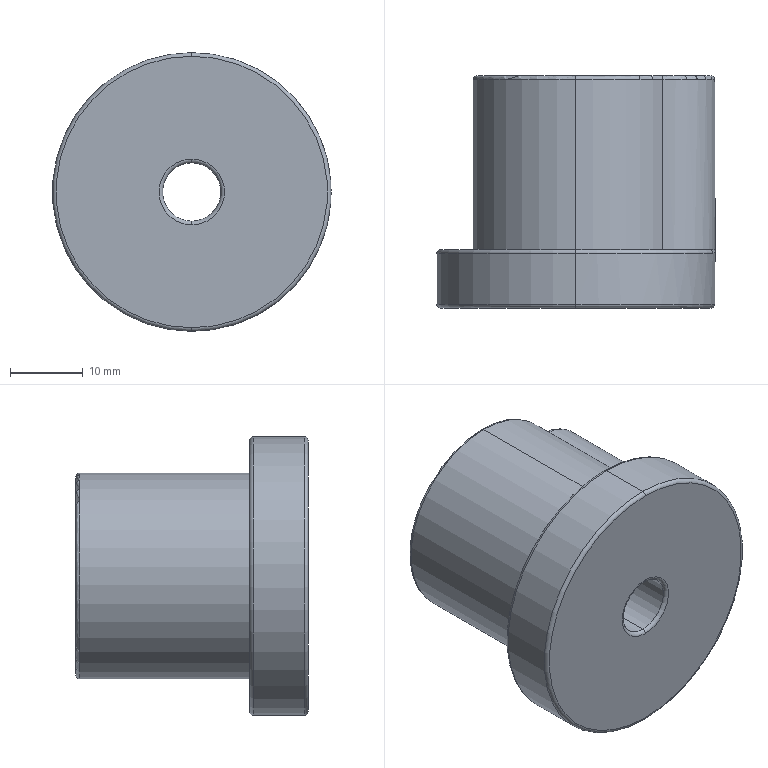Component | SolidWorks | Workpiece-1 | 1 solid | 26 faces | box 38.21 x 31.82 x 38.21 mm | volume 23902 mm3 | torus 13 | cylinder 8 | plane 3 | spline 2 | commonest cylinder face diameters 28.21 x3 38.21 x2 8 x2 15 x1 | material 45
STEP:
#1=COLOUR_RGB('',0.7922,0.8196,0.9333);
#2=FILL_AREA_STYLE_COLOUR('',#1);
#3=FILL_AREA_STYLE('',(#2));
#4=SURFACE_STYLE_FILL_AREA(#3);
#5=SURFACE_SIDE_STYLE('',(#4));
#6=SURFACE_STYLE_USAGE(.BOTH.,#5);
#7=PRESENTATION_STYLE_ASSIGNMENT((#6));
#8=CARTESIAN_POINT('',(-14.62,-0.1144,42.544));
#9=VERTEX_POINT('',#8);
#10=CARTESIAN_POINT('',(-13.9,-0.1144,41.945));
#11=VERTEX_POINT('',#10);
#12=CARTESIAN_POINT('',(-14.62,-0.1144,41.811));
#13=DIRECTION('',(0.,1.,0.));
#14=DIRECTION('',(-0.,0.,-1.));
#15=AXIS2_PLACEMENT_3D('',#12,#13,#14);
#16=CIRCLE('',#15,0.7325);
#17=EDGE_CURVE('',#9,#11,#16,.T.);
#18=ORIENTED_EDGE('',*,*,#17,.F.);
#19=CARTESIAN_POINT('',(-14.62,-0.1341,42.563));
#20=VERTEX_POINT('',#19);
#21=CARTESIAN_POINT('',(-14.62,-0.1341,42.544));
#22=DIRECTION('',(1.,0.,-0.));
#23=DIRECTION('',(0.,0.,-1.));
#24=AXIS2_PLACEMENT_3D('',#21,#22,#23);
#25=CIRCLE('',#24,0.01969);
#26=EDGE_CURVE('',#9,#20,#25,.T.);
#27=ORIENTED_EDGE('',*,*,#26,.T.);
#28=CARTESIAN_POINT('',(-13.881,-0.1341,41.948));
#29=VERTEX_POINT('',#28);
#30=CARTESIAN_POINT('',(-14.62,-0.1341,41.811));
#31=DIRECTION('',(0.,-1.,0.));
#32=DIRECTION('',(0.,0.,-1.));
#33=AXIS2_PLACEMENT_3D('',#30,#31,#32);
#34=CIRCLE('',#33,0.7522);
#35=EDGE_CURVE('',#29,#20,#34,.T.);
#36=ORIENTED_EDGE('',*,*,#35,.F.);
#37=CARTESIAN_POINT('',(-13.9,-0.1341,41.945));
#38=DIRECTION('',(0.1825,0.,-0.9832));
#39=DIRECTION('',(-0.9832,0.,-0.1825));
#40=AXIS2_PLACEMENT_3D('',#37,#38,#39);
#41=CIRCLE('',#40,0.01969);
#42=EDGE_CURVE('',#11,#29,#41,.T.);
#43=ORIENTED_EDGE('',*,*,#42,.F.);
#44=EDGE_LOOP('',(#18,#27,#36,#43));
#45=FACE_OUTER_BOUND('',#44,.T.);
#46=CARTESIAN_POINT('',(-14.62,-0.1341,41.811));
#47=DIRECTION('',(0.,-1.,0.));
#48=DIRECTION('',(0.,0.,-1.));
#49=AXIS2_PLACEMENT_3D('',#46,#47,#48);
#50=TOROIDAL_SURFACE('',#49,0.7325,0.01969);
#51=ADVANCED_FACE('',(#45),#50,.T.);
#52=ORIENTED_EDGE('',*,*,#26,.F.);
#53=CARTESIAN_POINT('',(-14.62,-0.1144,41.079));
#54=VERTEX_POINT('',#53);
#55=CARTESIAN_POINT('',(-14.62,-0.1144,41.811));
#56=DIRECTION('',(0.,1.,0.));
#57=DIRECTION('',(0.,0.,-1.));
#58=AXIS2_PLACEMENT_3D('',#55,#56,#57);
#59=CIRCLE('',#58,0.7325);
#60=EDGE_CURVE('',#54,#9,#59,.T.);
#61=ORIENTED_EDGE('',*,*,#60,.F.);
#62=CARTESIAN_POINT('',(-14.62,-0.1341,41.059));
#63=VERTEX_POINT('',#62);
#64=CARTESIAN_POINT('',(-14.62,-0.1341,41.079));
#65=DIRECTION('',(-1.,0.,0.));
#66=DIRECTION('',(0.,0.,1.));
#67=AXIS2_PLACEMENT_3D('',#64,#65,#66);
#68=CIRCLE('',#67,0.01969);
#69=EDGE_CURVE('',#54,#63,#68,.T.);
#70=ORIENTED_EDGE('',*,*,#69,.T.);
#71=CARTESIAN_POINT('',(-14.62,-0.1341,41.811));
#72=DIRECTION('',(0.,-1.,0.));
#73=DIRECTION('',(0.,0.,-1.));
#74=AXIS2_PLACEMENT_3D('',#71,#72,#73);
#75=CIRCLE('',#74,0.7522);
#76=EDGE_CURVE('',#20,#63,#75,.T.);
#77=ORIENTED_EDGE('',*,*,#76,.F.);
#78=EDGE_LOOP('',(#52,#61,#70,#77));
#79=FACE_OUTER_BOUND('',#78,.T.);
#80=CARTESIAN_POINT('',(-14.62,-0.1341,41.811));
#81=DIRECTION('',(0.,-1.,0.));
#82=DIRECTION('',(0.,0.,-1.));
#83=AXIS2_PLACEMENT_3D('',#80,#81,#82);
#84=TOROIDAL_SURFACE('',#83,0.7325,0.01969);
#85=ADVANCED_FACE('',(#79),#84,.T.);
#86=CARTESIAN_POINT('',(-14.62,0.8037,41.256));
#87=VERTEX_POINT('',#86);
#88=CARTESIAN_POINT('',(-14.15,0.8037,41.516));
#89=VERTEX_POINT('',#88);
#90=CARTESIAN_POINT('',(-14.62,0.8037,41.811));
#91=DIRECTION('',(0.,-1.,0.));
#92=DIRECTION('',(-0.,0.,1.));
#93=AXIS2_PLACEMENT_3D('',#90,#91,#92);
#94=CIRCLE('',#93,0.5553);
#95=EDGE_CURVE('',#87,#89,#94,.T.);
#96=ORIENTED_EDGE('',*,*,#95,.F.);
#97=CARTESIAN_POINT('',(-14.62,0.8234,41.275));
#98=VERTEX_POINT('',#97);
#99=CARTESIAN_POINT('',(-14.62,0.8037,41.275));
#100=DIRECTION('',(1.,0.,0.));
#101=DIRECTION('',(0.,0.,-1.));
#102=AXIS2_PLACEMENT_3D('',#99,#100,#101);
#103=CIRCLE('',#102,0.01969);
#104=EDGE_CURVE('',#87,#98,#103,.T.);
#105=ORIENTED_EDGE('',*,*,#104,.T.);
#106=CARTESIAN_POINT('',(-14.161,0.8234,41.535));
#107=VERTEX_POINT('',#106);
#108=CARTESIAN_POINT('',(-14.62,0.8234,41.811));
#109=DIRECTION('',(0.,1.,0.));
#110=DIRECTION('',(0.,0.,1.));
#111=AXIS2_PLACEMENT_3D('',#108,#109,#110);
#112=CIRCLE('',#111,0.5356);
#113=EDGE_CURVE('',#107,#98,#112,.T.);
#114=ORIENTED_EDGE('',*,*,#113,.F.);
#115=CARTESIAN_POINT('',(-14.15,0.8037,41.516));
#116=CARTESIAN_POINT('',(-14.15,0.8093,41.516));
#117=CARTESIAN_POINT('',(-14.151,0.8146,41.518));
#118=CARTESIAN_POINT('',(-14.156,0.8216,41.526));
#119=CARTESIAN_POINT('',(-14.158,0.8234,41.531));
#120=CARTESIAN_POINT('',(-14.161,0.8234,41.535));
#121=B_SPLINE_CURVE_WITH_KNOTS('',3,(#115,#116,#117,#118,#119,#120),.UNSPECIFIED.,.F.,.F.,(4,2,4),(0.,0.0004181,0.0008363),.UNSPECIFIED.);
#122=EDGE_CURVE('',#89,#107,#121,.T.);
#123=ORIENTED_EDGE('',*,*,#122,.F.);
#124=EDGE_LOOP('',(#96,#105,#114,#123));
#125=FACE_OUTER_BOUND('',#124,.T.);
#126=CARTESIAN_POINT('',(-14.62,0.8037,41.811));
#127=DIRECTION('',(0.,1.,0.));
#128=DIRECTION('',(0.,0.,1.));
#129=AXIS2_PLACEMENT_3D('',#126,#127,#128);
#130=TOROIDAL_SURFACE('',#129,0.5356,0.01969);
#131=ADVANCED_FACE('',(#125),#130,.T.);
#132=ORIENTED_EDGE('',*,*,#104,.F.);
#133=CARTESIAN_POINT('',(-14.62,0.8037,42.366));
#134=VERTEX_POINT('',#133);
#135=CARTESIAN_POINT('',(-14.62,0.8037,41.811));
#136=DIRECTION('',(0.,-1.,0.));
#137=DIRECTION('',(0.,0.,1.));
#138=AXIS2_PLACEMENT_3D('',#135,#136,#137);
#139=CIRCLE('',#138,0.5553);
#140=EDGE_CURVE('',#134,#87,#139,.T.);
#141=ORIENTED_EDGE('',*,*,#140,.F.);
#142=CARTESIAN_POINT('',(-14.62,0.8234,42.347));
#143=VERTEX_POINT('',#142);
#144=CARTESIAN_POINT('',(-14.62,0.8037,42.347));
#145=DIRECTION('',(-1.,0.,0.));
#146=DIRECTION('',(0.,0.,1.));
#147=AXIS2_PLACEMENT_3D('',#144,#145,#146);
#148=CIRCLE('',#147,0.01969);
#149=EDGE_CURVE('',#134,#143,#148,.T.);
#150=ORIENTED_EDGE('',*,*,#149,.T.);
#151=CARTESIAN_POINT('',(-14.62,0.8234,41.811));
#152=DIRECTION('',(0.,1.,0.));
#153=DIRECTION('',(0.,0.,1.));
#154=AXIS2_PLACEMENT_3D('',#151,#152,#153);
#155=CIRCLE('',#154,0.5356);
#156=EDGE_CURVE('',#98,#143,#155,.T.);
#157=ORIENTED_EDGE('',*,*,#156,.F.);
#158=EDGE_LOOP('',(#132,#141,#150,#157));
#159=FACE_OUTER_BOUND('',#158,.T.);
#160=CARTESIAN_POINT('',(-14.62,0.8037,41.811));
#161=DIRECTION('',(0.,1.,0.));
#162=DIRECTION('',(0.,0.,1.));
#163=AXIS2_PLACEMENT_3D('',#160,#161,#162);
#164=TOROIDAL_SURFACE('',#163,0.5356,0.01969);
#165=ADVANCED_FACE('',(#159),#164,.T.);
#166=CARTESIAN_POINT('',(-14.62,0.8234,41.634));
#167=VERTEX_POINT('',#166);
#168=CARTESIAN_POINT('',(-14.62,0.8234,41.988));
#169=VERTEX_POINT('',#168);
#170=CARTESIAN_POINT('',(-14.62,0.8234,41.811));
#171=DIRECTION('',(0.,-1.,0.));
#172=DIRECTION('',(0.,0.,1.));
#173=AXIS2_PLACEMENT_3D('',#170,#171,#172);
#174=CIRCLE('',#173,0.1772);
#175=EDGE_CURVE('',#167,#169,#174,.T.);
#176=ORIENTED_EDGE('',*,*,#175,.F.);
#177=CARTESIAN_POINT('',(-14.62,0.8037,41.654));
#178=VERTEX_POINT('',#177);
#179=CARTESIAN_POINT('',(-14.62,0.8037,41.634));
#180=DIRECTION('',(1.,0.,0.));
#181=DIRECTION('',(0.,0.,-1.));
#182=AXIS2_PLACEMENT_3D('',#179,#180,#181);
#183=CIRCLE('',#182,0.01969);
#184=EDGE_CURVE('',#167,#178,#183,.T.);
#185=ORIENTED_EDGE('',*,*,#184,.T.);
#186=CARTESIAN_POINT('',(-14.62,0.8037,41.969));
#187=VERTEX_POINT('',#186);
#188=CARTESIAN_POINT('',(-14.62,0.8037,41.811));
#189=DIRECTION('',(0.,1.,0.));
#190=DIRECTION('',(0.,0.,1.));
#191=AXIS2_PLACEMENT_3D('',#188,#189,#190);
#192=CIRCLE('',#191,0.1575);
#193=EDGE_CURVE('',#187,#178,#192,.T.);
#194=ORIENTED_EDGE('',*,*,#193,.F.);
#195=CARTESIAN_POINT('',(-14.62,0.8037,41.988));
#196=DIRECTION('',(-1.,0.,0.));
#197=DIRECTION('',(0.,0.,1.));
#198=AXIS2_PLACEMENT_3D('',#195,#196,#197);
#199=CIRCLE('',#198,0.01969);
#200=EDGE_CURVE('',#169,#187,#199,.T.);
#201=ORIENTED_EDGE('',*,*,#200,.F.);
#202=EDGE_LOOP('',(#176,#185,#194,#201));
#203=FACE_OUTER_BOUND('',#202,.T.);
#204=CARTESIAN_POINT('',(-14.62,0.8037,41.811));
#205=DIRECTION('',(0.,1.,0.));
#206=DIRECTION('',(0.,0.,1.));
#207=AXIS2_PLACEMENT_3D('',#204,#205,#206);
#208=TOROIDAL_SURFACE('',#207,0.1772,0.01969);
#209=ADVANCED_FACE('',(#203),#208,.T.);
#210=CARTESIAN_POINT('',(-14.62,-0.4097,42.563));
#211=VERTEX_POINT('',#210);
#212=CARTESIAN_POINT('',(-14.62,-0.4097,41.059));
#213=VERTEX_POINT('',#212);
#214=CARTESIAN_POINT('',(-14.62,-0.4097,41.811));
#215=DIRECTION('',(0.,1.,0.));
#216=DIRECTION('',(0.,0.,-1.));
#217=AXIS2_PLACEMENT_3D('',#214,#215,#216);
#218=CIRCLE('',#217,0.7522);
#219=EDGE_CURVE('',#211,#213,#218,.T.);
#220=ORIENTED_EDGE('',*,*,#219,.F.);
#221=CARTESIAN_POINT('',(-14.62,-0.4293,42.544));
#222=VERTEX_POINT('',#221);
#223=CARTESIAN_POINT('',(-14.62,-0.4097,42.544));
#224=DIRECTION('',(1.,0.,-0.));
#225=DIRECTION('',(0.,0.,-1.));
#226=AXIS2_PLACEMENT_3D('',#223,#224,#225);
#227=CIRCLE('',#226,0.01969);
#228=EDGE_CURVE('',#211,#222,#227,.T.);
#229=ORIENTED_EDGE('',*,*,#228,.T.);
#230=CARTESIAN_POINT('',(-14.62,-0.4293,41.079));
#231=VERTEX_POINT('',#230);
#232=CARTESIAN_POINT('',(-14.62,-0.4293,41.811));
#233=DIRECTION('',(0.,-1.,0.));
#234=DIRECTION('',(0.,0.,-1.));
#235=AXIS2_PLACEMENT_3D('',#232,#233,#234);
#236=CIRCLE('',#235,0.7325);
#237=EDGE_CURVE('',#231,#222,#236,.T.);
#238=ORIENTED_EDGE('',*,*,#237,.F.);
#239=CARTESIAN_POINT('',(-14.62,-0.4097,41.079));
#240=DIRECTION('',(-1.,0.,0.));
#241=DIRECTION('',(0.,0.,1.));
#242=AXIS2_PLACEMENT_3D('',#239,#240,#241);
#243=CIRCLE('',#242,0.01969);
#244=EDGE_CURVE('',#213,#231,#243,.T.);
#245=ORIENTED_EDGE('',*,*,#244,.F.);
#246=EDGE_LOOP('',(#220,#229,#238,#245));
#247=FACE_OUTER_BOUND('',#246,.T.);
#248=CARTESIAN_POINT('',(-14.62,-0.4097,41.811));
#249=DIRECTION('',(0.,-1.,0.));
#250=DIRECTION('',(0.,0.,-1.));
#251=AXIS2_PLACEMENT_3D('',#248,#249,#250);
#252=TOROIDAL_SURFACE('',#251,0.7325,0.01969);
#253=ADVANCED_FACE('',(#247),#252,.T.);
#254=CARTESIAN_POINT('',(-14.62,-0.4293,41.988));
#255=VERTEX_POINT('',#254);
#256=CARTESIAN_POINT('',(-14.62,-0.4293,41.634));
#257=VERTEX_POINT('',#256);
#258=CARTESIAN_POINT('',(-14.62,-0.4293,41.811));
#259=DIRECTION('',(0.,1.,0.));
#260=DIRECTION('',(0.,0.,-1.));
#261=AXIS2_PLACEMENT_3D('',#258,#259,#260);
#262=CIRCLE('',#261,0.1772);
#263=EDGE_CURVE('',#255,#257,#262,.T.);
#264=ORIENTED_EDGE('',*,*,#263,.F.);
#265=CARTESIAN_POINT('',(-14.62,-0.4097,41.969));
#266=VERTEX_POINT('',#265);
#267=CARTESIAN_POINT('',(-14.62,-0.4097,41.988));
#268=DIRECTION('',(1.,0.,-0.));
#269=DIRECTION('',(0.,0.,-1.));
#270=AXIS2_PLACEMENT_3D('',#267,#268,#269);
#271=CIRCLE('',#270,0.01969);
#272=EDGE_CURVE('',#255,#266,#271,.T.);
#273=ORIENTED_EDGE('',*,*,#272,.T.);
#274=CARTESIAN_POINT('',(-14.62,-0.4097,41.654));
#275=VERTEX_POINT('',#274);
#276=CARTESIAN_POINT('',(-14.62,-0.4097,41.811));
#277=DIRECTION('',(0.,-1.,0.));
#278=DIRECTION('',(0.,0.,-1.));
#279=AXIS2_PLACEMENT_3D('',#276,#277,#278);
#280=CIRCLE('',#279,0.1575);
#281=EDGE_CURVE('',#275,#266,#280,.T.);
#282=ORIENTED_EDGE('',*,*,#281,.F.);
#283=CARTESIAN_POINT('',(-14.62,-0.4097,41.634));
#284=DIRECTION('',(-1.,0.,0.));
#285=DIRECTION('',(0.,0.,1.));
#286=AXIS2_PLACEMENT_3D('',#283,#284,#285);
#287=CIRCLE('',#286,0.01969);
#288=EDGE_CURVE('',#257,#275,#287,.T.);
#289=ORIENTED_EDGE('',*,*,#288,.F.);
#290=EDGE_LOOP('',(#264,#273,#282,#289));
#291=FACE_OUTER_BOUND('',#290,.T.);
#292=CARTESIAN_POINT('',(-14.62,-0.4097,41.811));
#293=DIRECTION('',(0.,-1.,0.));
#294=DIRECTION('',(0.,0.,-1.));
#295=AXIS2_PLACEMENT_3D('',#292,#293,#294);
#296=TOROIDAL_SURFACE('',#295,0.1772,0.01969);
#297=ADVANCED_FACE('',(#291),#296,.T.);
#298=ORIENTED_EDGE('',*,*,#219,.T.);
#299=CARTESIAN_POINT('',(-14.62,-0.4293,41.059));
#300=DIRECTION('',(0.,1.,0.));
#301=VECTOR('',#300,39.37);
#302=LINE('',#299,#301);
#303=EDGE_CURVE('',#213,#63,#302,.T.);
#304=ORIENTED_EDGE('',*,*,#303,.T.);
#305=CARTESIAN_POINT('',(-13.881,-0.1341,41.674));
#306=VERTEX_POINT('',#305);
#307=CARTESIAN_POINT('',(-14.62,-0.1341,41.811));
#308=DIRECTION('',(0.,-1.,0.));
#309=DIRECTION('',(0.,0.,-1.));
#310=AXIS2_PLACEMENT_3D('',#307,#308,#309);
#311=CIRCLE('',#310,0.7522);
#312=EDGE_CURVE('',#63,#306,#311,.T.);
#313=ORIENTED_EDGE('',*,*,#312,.T.);
#314=CARTESIAN_POINT('',(-13.868,-0.1144,41.811));
#315=VERTEX_POINT('',#314);
#316=CARTESIAN_POINT('',(-13.881,-0.1341,41.674));
#317=CARTESIAN_POINT('',(-13.879,-0.1341,41.685));
#318=CARTESIAN_POINT('',(-13.877,-0.1333,41.697));
#319=CARTESIAN_POINT('',(-13.874,-0.1309,41.72));
#320=CARTESIAN_POINT('',(-13.872,-0.1293,41.731));
#321=CARTESIAN_POINT('',(-13.87,-0.1256,41.754));
#322=CARTESIAN_POINT('',(-13.87,-0.1235,41.765));
#323=CARTESIAN_POINT('',(-13.869,-0.1191,41.788));
#324=CARTESIAN_POINT('',(-13.868,-0.1167,41.8));
#325=CARTESIAN_POINT('',(-13.868,-0.1144,41.811));
#326=B_SPLINE_CURVE_WITH_KNOTS('',3,(#316,#317,#318,#319,#320,#321,#322,#323,#324,#325),.UNSPECIFIED.,.F.,.F.,(4,2,2,2,4),(0.,0.0008842,0.001768,0.002653,0.003537),.UNSPECIFIED.);
#327=EDGE_CURVE('',#306,#315,#326,.T.);
#328=ORIENTED_EDGE('',*,*,#327,.T.);
#329=CARTESIAN_POINT('',(-13.868,-0.1144,41.811));
#330=CARTESIAN_POINT('',(-13.868,-0.1191,41.834));
#331=CARTESIAN_POINT('',(-13.869,-0.1238,41.857));
#332=CARTESIAN_POINT('',(-13.872,-0.1293,41.891));
#333=CARTESIAN_POINT('',(-13.874,-0.131,41.902));
#334=CARTESIAN_POINT('',(-13.877,-0.1333,41.925));
#335=CARTESIAN_POINT('',(-13.879,-0.1341,41.937));
#336=CARTESIAN_POINT('',(-13.881,-0.1341,41.948));
#337=B_SPLINE_CURVE_WITH_KNOTS('',3,(#329,#330,#331,#332,#333,#334,#335,#336),.UNSPECIFIED.,.F.,.F.,(4,2,2,4),(-0.00002194,0.001756,0.002645,0.003534),.UNSPECIFIED.);
#338=EDGE_CURVE('',#315,#29,#337,.T.);
#339=ORIENTED_EDGE('',*,*,#338,.T.);
#340=ORIENTED_EDGE('',*,*,#35,.T.);
#341=CARTESIAN_POINT('',(-14.62,-0.4293,42.563));
#342=DIRECTION('',(0.,1.,0.));
#343=VECTOR('',#342,39.37);
#344=LINE('',#341,#343);
#345=EDGE_CURVE('',#211,#20,#344,.T.);
#346=ORIENTED_EDGE('',*,*,#345,.F.);
#347=EDGE_LOOP('',(#298,#304,#313,#328,#339,#340,#346));
#348=FACE_OUTER_BOUND('',#347,.T.);
#349=CARTESIAN_POINT('',(-14.62,-0.4293,41.811));
#350=DIRECTION('',(0.,1.,0.));
#351=DIRECTION('',(0.,0.,1.));
#352=AXIS2_PLACEMENT_3D('',#349,#350,#351);
#353=CYLINDRICAL_SURFACE('',#352,0.7522);
#354=ADVANCED_FACE('',(#348),#353,.T.);
#355=CARTESIAN_POINT('',(-14.62,0.8037,41.811));
#356=DIRECTION('',(0.,1.,0.));
#357=DIRECTION('',(0.,0.,1.));
#358=AXIS2_PLACEMENT_3D('',#355,#356,#357);
#359=CIRCLE('',#358,0.1575);
#360=EDGE_CURVE('',#178,#187,#359,.T.);
#361=ORIENTED_EDGE('',*,*,#360,.T.);
#362=CARTESIAN_POINT('',(-14.62,0.8234,41.969));
#363=DIRECTION('',(0.,-1.,0.));
#364=VECTOR('',#363,39.37);
#365=LINE('',#362,#364);
#366=EDGE_CURVE('',#187,#266,#365,.T.);
#367=ORIENTED_EDGE('',*,*,#366,.T.);
#368=CARTESIAN_POINT('',(-14.62,-0.4097,41.811));
#369=DIRECTION('',(0.,-1.,0.));
#370=DIRECTION('',(0.,0.,-1.));
#371=AXIS2_PLACEMENT_3D('',#368,#369,#370);
#372=CIRCLE('',#371,0.1575);
#373=EDGE_CURVE('',#266,#275,#372,.T.);
#374=ORIENTED_EDGE('',*,*,#373,.T.);
#375=CARTESIAN_POINT('',(-14.62,0.8234,41.654));
#376=DIRECTION('',(0.,-1.,0.));
#377=VECTOR('',#376,39.37);
#378=LINE('',#375,#377);
#379=EDGE_CURVE('',#178,#275,#378,.T.);
#380=ORIENTED_EDGE('',*,*,#379,.F.);
#381=EDGE_LOOP('',(#361,#367,#374,#380));
#382=FACE_OUTER_BOUND('',#381,.T.);
#383=CARTESIAN_POINT('',(-14.62,0.8234,41.811));
#384=DIRECTION('',(0.,-1.,0.));
#385=DIRECTION('',(0.,0.,-1.));
#386=AXIS2_PLACEMENT_3D('',#383,#384,#385);
#387=CYLINDRICAL_SURFACE('',#386,0.1575);
#388=ADVANCED_FACE('',(#382),#387,.F.);
#389=CARTESIAN_POINT('',(-14.15,0.8037,42.106));
#390=VERTEX_POINT('',#389);
#391=CARTESIAN_POINT('',(-14.62,0.8037,41.811));
#392=DIRECTION('',(0.,-1.,0.));
#393=DIRECTION('',(-0.,0.,1.));
#394=AXIS2_PLACEMENT_3D('',#391,#392,#393);
#395=CIRCLE('',#394,0.5553);
#396=EDGE_CURVE('',#390,#134,#395,.T.);
#397=ORIENTED_EDGE('',*,*,#396,.T.);
#398=CARTESIAN_POINT('',(-14.62,-0.1144,42.366));
#399=VERTEX_POINT('',#398);
#400=CARTESIAN_POINT('',(-14.62,0.8234,42.366));
#401=DIRECTION('',(0.,-1.,0.));
#402=VECTOR('',#401,39.37);
#403=LINE('',#400,#402);
#404=EDGE_CURVE('',#134,#399,#403,.T.);
#405=ORIENTED_EDGE('',*,*,#404,.T.);
#406=CARTESIAN_POINT('',(-14.15,-0.1144,42.106));
#407=VERTEX_POINT('',#406);
#408=CARTESIAN_POINT('',(-14.62,-0.1144,41.811));
#409=DIRECTION('',(0.,1.,0.));
#410=DIRECTION('',(0.,0.,1.));
#411=AXIS2_PLACEMENT_3D('',#408,#409,#410);
#412=CIRCLE('',#411,0.5553);
#413=EDGE_CURVE('',#399,#407,#412,.T.);
#414=ORIENTED_EDGE('',*,*,#413,.T.);
#415=CARTESIAN_POINT('',(-14.15,-0.7681,42.106));
#416=DIRECTION('',(0.,1.,0.));
#417=VECTOR('',#416,39.37);
#418=LINE('',#415,#417);
#419=EDGE_CURVE('',#407,#390,#418,.T.);
#420=ORIENTED_EDGE('',*,*,#419,.T.);
#421=EDGE_LOOP('',(#397,#405,#414,#420));
#422=FACE_OUTER_BOUND('',#421,.T.);
#423=CARTESIAN_POINT('',(-14.62,0.8234,41.811));
#424=DIRECTION('',(0.,-1.,0.));
#425=DIRECTION('',(0.,0.,-1.));
#426=AXIS2_PLACEMENT_3D('',#423,#424,#425);
#427=CYLINDRICAL_SURFACE('',#426,0.5553);
#428=ADVANCED_FACE('',(#422),#427,.T.);
#429=ORIENTED_EDGE('',*,*,#404,.F.);
#430=ORIENTED_EDGE('',*,*,#140,.T.);
#431=CARTESIAN_POINT('',(-14.62,-0.1144,41.256));
#432=VERTEX_POINT('',#431);
#433=CARTESIAN_POINT('',(-14.62,0.8234,41.256));
#434=DIRECTION('',(0.,-1.,0.));
#435=VECTOR('',#434,39.37);
#436=LINE('',#433,#435);
#437=EDGE_CURVE('',#87,#432,#436,.T.);
#438=ORIENTED_EDGE('',*,*,#437,.T.);
#439=CARTESIAN_POINT('',(-14.62,-0.1144,41.811));
#440=DIRECTION('',(0.,1.,0.));
#441=DIRECTION('',(0.,0.,1.));
#442=AXIS2_PLACEMENT_3D('',#439,#440,#441);
#443=CIRCLE('',#442,0.5553);
#444=EDGE_CURVE('',#432,#399,#443,.T.);
#445=ORIENTED_EDGE('',*,*,#444,.T.);
#446=EDGE_LOOP('',(#429,#430,#438,#445));
#447=FACE_OUTER_BOUND('',#446,.T.);
#448=CARTESIAN_POINT('',(-14.62,0.8234,41.811));
#449=DIRECTION('',(0.,-1.,0.));
#450=DIRECTION('',(0.,0.,-1.));
#451=AXIS2_PLACEMENT_3D('',#448,#449,#450);
#452=CYLINDRICAL_SURFACE('',#451,0.5553);
#453=ADVANCED_FACE('',(#447),#452,.T.);
#454=CARTESIAN_POINT('',(-14.62,0.8234,41.811));
#455=DIRECTION('',(0.,-1.,0.));
#456=DIRECTION('',(0.,0.,1.));
#457=AXIS2_PLACEMENT_3D('',#454,#455,#456);
#458=CIRCLE('',#457,0.1772);
#459=EDGE_CURVE('',#169,#167,#458,.T.);
#460=ORIENTED_EDGE('',*,*,#459,.T.);
#461=ORIENTED_EDGE('',*,*,#175,.T.);
#462=EDGE_LOOP('',(#460,#461));
#463=FACE_BOUND('',#462,.T.);
#464=ORIENTED_EDGE('',*,*,#113,.T.);
#465=ORIENTED_EDGE('',*,*,#156,.T.);
#466=CARTESIAN_POINT('',(-14.161,0.8234,42.087));
#467=VERTEX_POINT('',#466);
#468=CARTESIAN_POINT('',(-14.62,0.8234,41.811));
#469=DIRECTION('',(0.,1.,0.));
#470=DIRECTION('',(0.,0.,1.));
#471=AXIS2_PLACEMENT_3D('',#468,#469,#470);
#472=CIRCLE('',#471,0.5356);
#473=EDGE_CURVE('',#143,#467,#472,.T.);
#474=ORIENTED_EDGE('',*,*,#473,.T.);
#475=CARTESIAN_POINT('',(-14.164,0.8234,41.811));
#476=DIRECTION('',(0.,1.,0.));
#477=DIRECTION('',(0.,0.,1.));
#478=AXIS2_PLACEMENT_3D('',#475,#476,#477);
#479=CIRCLE('',#478,0.2756);
#480=EDGE_CURVE('',#467,#107,#479,.T.);
#481=ORIENTED_EDGE('',*,*,#480,.T.);
#482=EDGE_LOOP('',(#464,#465,#474,#481));
#483=FACE_OUTER_BOUND('',#482,.T.);
#484=CARTESIAN_POINT('',(-14.62,0.8234,41.811));
#485=DIRECTION('',(0.,1.,0.));
#486=DIRECTION('',(0.,0.,1.));
#487=AXIS2_PLACEMENT_3D('',#484,#485,#486);
#488=PLANE('',#487);
#489=ADVANCED_FACE('',(#463,#483),#488,.T.);
#490=ORIENTED_EDGE('',*,*,#437,.F.);
#491=ORIENTED_EDGE('',*,*,#95,.T.);
#492=CARTESIAN_POINT('',(-14.15,-0.1144,41.516));
#493=VERTEX_POINT('',#492);
#494=CARTESIAN_POINT('',(-14.15,-0.7681,41.516));
#495=DIRECTION('',(0.,1.,0.));
#496=VECTOR('',#495,39.37);
#497=LINE('',#494,#496);
#498=EDGE_CURVE('',#493,#89,#497,.T.);
#499=ORIENTED_EDGE('',*,*,#498,.F.);
#500=CARTESIAN_POINT('',(-14.62,-0.1144,41.811));
#501=DIRECTION('',(0.,1.,0.));
#502=DIRECTION('',(0.,0.,1.));
#503=AXIS2_PLACEMENT_3D('',#500,#501,#502);
#504=CIRCLE('',#503,0.5553);
#505=EDGE_CURVE('',#493,#432,#504,.T.);
#506=ORIENTED_EDGE('',*,*,#505,.T.);
#507=EDGE_LOOP('',(#490,#491,#499,#506));
#508=FACE_OUTER_BOUND('',#507,.T.);
#509=CARTESIAN_POINT('',(-14.62,0.8234,41.811));
#510=DIRECTION('',(0.,-1.,0.));
#511=DIRECTION('',(0.,0.,-1.));
#512=AXIS2_PLACEMENT_3D('',#509,#510,#511);
#513=CYLINDRICAL_SURFACE('',#512,0.5553);
#514=ADVANCED_FACE('',(#508),#513,.T.);
#515=ORIENTED_EDGE('',*,*,#366,.F.);
#516=ORIENTED_EDGE('',*,*,#193,.T.);
#517=ORIENTED_EDGE('',*,*,#379,.T.);
#518=ORIENTED_EDGE('',*,*,#281,.T.);
#519=EDGE_LOOP('',(#515,#516,#517,#518));
#520=FACE_OUTER_BOUND('',#519,.T.);
#521=CARTESIAN_POINT('',(-14.62,0.8234,41.811));
#522=DIRECTION('',(0.,-1.,0.));
#523=DIRECTION('',(0.,0.,-1.));
#524=AXIS2_PLACEMENT_3D('',#521,#522,#523);
#525=CYLINDRICAL_SURFACE('',#524,0.1575);
#526=ADVANCED_FACE('',(#520),#525,.F.);
#527=CARTESIAN_POINT('',(-14.62,-0.4293,41.811));
#528=DIRECTION('',(0.,1.,0.));
#529=DIRECTION('',(0.,0.,-1.));
#530=AXIS2_PLACEMENT_3D('',#527,#528,#529);
#531=CIRCLE('',#530,0.1772);
#532=EDGE_CURVE('',#257,#255,#531,.T.);
#533=ORIENTED_EDGE('',*,*,#532,.T.);
#534=ORIENTED_EDGE('',*,*,#263,.T.);
#535=EDGE_LOOP('',(#533,#534));
#536=FACE_BOUND('',#535,.T.);
#537=ORIENTED_EDGE('',*,*,#237,.T.);
#538=CARTESIAN_POINT('',(-14.62,-0.4293,41.811));
#539=DIRECTION('',(0.,-1.,0.));
#540=DIRECTION('',(0.,0.,-1.));
#541=AXIS2_PLACEMENT_3D('',#538,#539,#540);
#542=CIRCLE('',#541,0.7325);
#543=EDGE_CURVE('',#222,#231,#542,.T.);
#544=ORIENTED_EDGE('',*,*,#543,.T.);
#545=EDGE_LOOP('',(#537,#544));
#546=FACE_OUTER_BOUND('',#545,.T.);
#547=CARTESIAN_POINT('',(-14.62,-0.4293,41.811));
#548=DIRECTION('',(0.,-1.,0.));
#549=DIRECTION('',(0.,0.,-1.));
#550=AXIS2_PLACEMENT_3D('',#547,#548,#549);
#551=PLANE('',#550);
#552=ADVANCED_FACE('',(#536,#546),#551,.T.);
#553=CARTESIAN_POINT('',(-13.9,-0.1144,41.677));
#554=VERTEX_POINT('',#553);
#555=CARTESIAN_POINT('',(-14.164,-0.1144,41.811));
#556=DIRECTION('',(0.,1.,0.));
#557=DIRECTION('',(0.,0.,-1.));
#558=AXIS2_PLACEMENT_3D('',#555,#556,#557);
#559=CIRCLE('',#558,0.2953);
#560=EDGE_CURVE('',#554,#493,#559,.T.);
#561=ORIENTED_EDGE('',*,*,#560,.F.);
#562=CARTESIAN_POINT('',(-14.62,-0.1144,41.811));
#563=DIRECTION('',(0.,1.,0.));
#564=DIRECTION('',(0.,0.,-1.));
#565=AXIS2_PLACEMENT_3D('',#562,#563,#564);
#566=CIRCLE('',#565,0.7325);
#567=EDGE_CURVE('',#554,#54,#566,.T.);
#568=ORIENTED_EDGE('',*,*,#567,.T.);
#569=ORIENTED_EDGE('',*,*,#60,.T.);
#570=ORIENTED_EDGE('',*,*,#17,.T.);
#571=CARTESIAN_POINT('',(-14.164,-0.1144,41.811));
#572=DIRECTION('',(0.,1.,0.));
#573=DIRECTION('',(0.,0.,-1.));
#574=AXIS2_PLACEMENT_3D('',#571,#572,#573);
#575=CIRCLE('',#574,0.2953);
#576=EDGE_CURVE('',#407,#11,#575,.T.);
#577=ORIENTED_EDGE('',*,*,#576,.F.);
#578=ORIENTED_EDGE('',*,*,#413,.F.);
#579=ORIENTED_EDGE('',*,*,#444,.F.);
#580=ORIENTED_EDGE('',*,*,#505,.F.);
#581=EDGE_LOOP('',(#561,#568,#569,#570,#577,#578,#579,#580));
#582=FACE_OUTER_BOUND('',#581,.T.);
#583=CARTESIAN_POINT('',(-14.62,-0.1144,41.811));
#584=DIRECTION('',(0.,-1.,0.));
#585=DIRECTION('',(0.,0.,-1.));
#586=AXIS2_PLACEMENT_3D('',#583,#584,#585);
#587=PLANE('',#586);
#588=ADVANCED_FACE('',(#582),#587,.F.);
#589=ORIENTED_EDGE('',*,*,#303,.F.);
#590=CARTESIAN_POINT('',(-14.62,-0.4097,41.811));
#591=DIRECTION('',(0.,1.,0.));
#592=DIRECTION('',(0.,0.,-1.));
#593=AXIS2_PLACEMENT_3D('',#590,#591,#592);
#594=CIRCLE('',#593,0.7522);
#595=EDGE_CURVE('',#213,#211,#594,.T.);
#596=ORIENTED_EDGE('',*,*,#595,.T.);
#597=ORIENTED_EDGE('',*,*,#345,.T.);
#598=ORIENTED_EDGE('',*,*,#76,.T.);
#599=EDGE_LOOP('',(#589,#596,#597,#598));
#600=FACE_OUTER_BOUND('',#599,.T.);
#601=CARTESIAN_POINT('',(-14.62,-0.4293,41.811));
#602=DIRECTION('',(0.,1.,0.));
#603=DIRECTION('',(0.,0.,1.));
#604=AXIS2_PLACEMENT_3D('',#601,#602,#603);
#605=CYLINDRICAL_SURFACE('',#604,0.7522);
#606=ADVANCED_FACE('',(#600),#605,.T.);
#607=ORIENTED_EDGE('',*,*,#498,.T.);
#608=CARTESIAN_POINT('',(-14.164,0.8037,41.811));
#609=DIRECTION('',(0.,-1.,0.));
#610=DIRECTION('',(0.,0.,1.));
#611=AXIS2_PLACEMENT_3D('',#608,#609,#610);
#612=CIRCLE('',#611,0.2953);
#613=EDGE_CURVE('',#89,#390,#612,.T.);
#614=ORIENTED_EDGE('',*,*,#613,.T.);
#615=ORIENTED_EDGE('',*,*,#419,.F.);
#616=ORIENTED_EDGE('',*,*,#576,.T.);
#617=CARTESIAN_POINT('',(-14.164,-0.1144,41.811));
#618=DIRECTION('',(0.,1.,0.));
#619=DIRECTION('',(-0.,0.,-1.));
#620=AXIS2_PLACEMENT_3D('',#617,#618,#619);
#621=CIRCLE('',#620,0.2953);
#622=EDGE_CURVE('',#11,#315,#621,.T.);
#623=ORIENTED_EDGE('',*,*,#622,.T.);
#624=CARTESIAN_POINT('',(-14.164,-0.1144,41.811));
#625=DIRECTION('',(0.,1.,0.));
#626=DIRECTION('',(-0.,0.,-1.));
#627=AXIS2_PLACEMENT_3D('',#624,#625,#626);
#628=CIRCLE('',#627,0.2953);
#629=EDGE_CURVE('',#315,#554,#628,.T.);
#630=ORIENTED_EDGE('',*,*,#629,.T.);
#631=ORIENTED_EDGE('',*,*,#560,.T.);
#632=EDGE_LOOP('',(#607,#614,#615,#616,#623,#630,#631));
#633=FACE_OUTER_BOUND('',#632,.T.);
#634=CARTESIAN_POINT('',(-14.164,-0.7681,41.811));
#635=DIRECTION('',(0.,1.,0.));
#636=DIRECTION('',(0.,0.,1.));
#637=AXIS2_PLACEMENT_3D('',#634,#635,#636);
#638=CYLINDRICAL_SURFACE('',#637,0.2953);
#639=ADVANCED_FACE('',(#633),#638,.T.);
#640=ORIENTED_EDGE('',*,*,#272,.F.);
#641=ORIENTED_EDGE('',*,*,#532,.F.);
#642=ORIENTED_EDGE('',*,*,#288,.T.);
#643=ORIENTED_EDGE('',*,*,#373,.F.);
#644=EDGE_LOOP('',(#640,#641,#642,#643));
#645=FACE_OUTER_BOUND('',#644,.T.);
#646=CARTESIAN_POINT('',(-14.62,-0.4097,41.811));
#647=DIRECTION('',(0.,-1.,0.));
#648=DIRECTION('',(0.,0.,-1.));
#649=AXIS2_PLACEMENT_3D('',#646,#647,#648);
#650=TOROIDAL_SURFACE('',#649,0.1772,0.01969);
#651=ADVANCED_FACE('',(#645),#650,.T.);
#652=ORIENTED_EDGE('',*,*,#228,.F.);
#653=ORIENTED_EDGE('',*,*,#595,.F.);
#654=ORIENTED_EDGE('',*,*,#244,.T.);
#655=ORIENTED_EDGE('',*,*,#543,.F.);
#656=EDGE_LOOP('',(#652,#653,#654,#655));
#657=FACE_OUTER_BOUND('',#656,.T.);
#658=CARTESIAN_POINT('',(-14.62,-0.4097,41.811));
#659=DIRECTION('',(0.,-1.,0.));
#660=DIRECTION('',(0.,0.,-1.));
#661=AXIS2_PLACEMENT_3D('',#658,#659,#660);
#662=TOROIDAL_SURFACE('',#661,0.7325,0.01969);
#663=ADVANCED_FACE('',(#657),#662,.T.);
#664=ORIENTED_EDGE('',*,*,#184,.F.);
#665=ORIENTED_EDGE('',*,*,#459,.F.);
#666=ORIENTED_EDGE('',*,*,#200,.T.);
#667=ORIENTED_EDGE('',*,*,#360,.F.);
#668=EDGE_LOOP('',(#664,#665,#666,#667));
#669=FACE_OUTER_BOUND('',#668,.T.);
#670=CARTESIAN_POINT('',(-14.62,0.8037,41.811));
#671=DIRECTION('',(0.,1.,0.));
#672=DIRECTION('',(0.,0.,1.));
#673=AXIS2_PLACEMENT_3D('',#670,#671,#672);
#674=TOROIDAL_SURFACE('',#673,0.1772,0.01969);
#675=ADVANCED_FACE('',(#669),#674,.T.);
#676=ORIENTED_EDGE('',*,*,#149,.F.);
#677=ORIENTED_EDGE('',*,*,#396,.F.);
#678=CARTESIAN_POINT('',(-14.161,0.8234,42.087));
#679=CARTESIAN_POINT('',(-14.158,0.8234,42.091));
#680=CARTESIAN_POINT('',(-14.156,0.8216,42.096));
#681=CARTESIAN_POINT('',(-14.151,0.8146,42.104));
#682=CARTESIAN_POINT('',(-14.15,0.8093,42.106));
#683=CARTESIAN_POINT('',(-14.15,0.8037,42.106));
#684=B_SPLINE_CURVE_WITH_KNOTS('',3,(#678,#679,#680,#681,#682,#683),.UNSPECIFIED.,.F.,.F.,(4,2,4),(-0.00000484,0.0004138,0.0008325),.UNSPECIFIED.);
#685=EDGE_CURVE('',#467,#390,#684,.T.);
#686=ORIENTED_EDGE('',*,*,#685,.F.);
#687=ORIENTED_EDGE('',*,*,#473,.F.);
#688=EDGE_LOOP('',(#676,#677,#686,#687));
#689=FACE_OUTER_BOUND('',#688,.T.);
#690=CARTESIAN_POINT('',(-14.62,0.8037,41.811));
#691=DIRECTION('',(0.,1.,0.));
#692=DIRECTION('',(0.,0.,1.));
#693=AXIS2_PLACEMENT_3D('',#690,#691,#692);
#694=TOROIDAL_SURFACE('',#693,0.5356,0.01969);
#695=ADVANCED_FACE('',(#689),#694,.T.);
#696=ORIENTED_EDGE('',*,*,#685,.T.);
#697=ORIENTED_EDGE('',*,*,#613,.F.);
#698=ORIENTED_EDGE('',*,*,#122,.T.);
#699=ORIENTED_EDGE('',*,*,#480,.F.);
#700=EDGE_LOOP('',(#696,#697,#698,#699));
#701=FACE_OUTER_BOUND('',#700,.T.);
#702=CARTESIAN_POINT('',(-14.164,0.8037,41.811));
#703=DIRECTION('',(0.,1.,0.));
#704=DIRECTION('',(0.,0.,1.));
#705=AXIS2_PLACEMENT_3D('',#702,#703,#704);
#706=TOROIDAL_SURFACE('',#705,0.2756,0.01969);
#707=ADVANCED_FACE('',(#701),#706,.T.);
#708=ORIENTED_EDGE('',*,*,#629,.F.);
#709=ORIENTED_EDGE('',*,*,#327,.F.);
#710=CARTESIAN_POINT('',(-13.9,-0.1341,41.677));
#711=DIRECTION('',(-0.1825,0.,-0.9832));
#712=DIRECTION('',(-0.9832,0.,0.1825));
#713=AXIS2_PLACEMENT_3D('',#710,#711,#712);
#714=CIRCLE('',#713,0.01969);
#715=EDGE_CURVE('',#554,#306,#714,.T.);
#716=ORIENTED_EDGE('',*,*,#715,.F.);
#717=EDGE_LOOP('',(#708,#709,#716));
#718=FACE_OUTER_BOUND('',#717,.T.);
#719=CARTESIAN_POINT('',(-13.9,-0.1144,41.677));
#720=CARTESIAN_POINT('',(-13.881,-0.1144,41.674));
#721=CARTESIAN_POINT('',(-13.881,-0.1341,41.674));
#722=CARTESIAN_POINT('',(-13.895,-0.1144,41.687));
#723=CARTESIAN_POINT('',(-13.879,-0.1173,41.684));
#724=CARTESIAN_POINT('',(-13.879,-0.1341,41.685));
#725=CARTESIAN_POINT('',(-13.891,-0.1144,41.697));
#726=CARTESIAN_POINT('',(-13.877,-0.1189,41.695));
#727=CARTESIAN_POINT('',(-13.877,-0.1333,41.697));
#728=CARTESIAN_POINT('',(-13.883,-0.1144,41.719));
#729=CARTESIAN_POINT('',(-13.874,-0.1204,41.718));
#730=CARTESIAN_POINT('',(-13.874,-0.131,41.72));
#731=CARTESIAN_POINT('',(-13.88,-0.1144,41.73));
#732=CARTESIAN_POINT('',(-13.873,-0.1204,41.729));
#733=CARTESIAN_POINT('',(-13.872,-0.1293,41.731));
#734=CARTESIAN_POINT('',(-13.871,-0.1144,41.763));
#735=CARTESIAN_POINT('',(-13.869,-0.1192,41.763));
#736=CARTESIAN_POINT('',(-13.869,-0.1238,41.765));
#737=CARTESIAN_POINT('',(-13.868,-0.1144,41.787));
#738=CARTESIAN_POINT('',(-13.868,-0.1167,41.788));
#739=CARTESIAN_POINT('',(-13.868,-0.1191,41.788));
#740=CARTESIAN_POINT('',(-13.868,-0.1144,41.811));
#741=CARTESIAN_POINT('',(-13.868,-0.1144,41.811));
#742=CARTESIAN_POINT('',(-13.868,-0.1144,41.811));
#743=(BOUNDED_SURFACE()B_SPLINE_SURFACE(3,2,((#719,#720,#721),(#722,#723,#724),(#725,#726,#727),(#728,#729,#730),(#731,#732,#733),(#734,#735,#736),(#737,#738,#739),(#740,#741,#742)),.UNSPECIFIED.,.F.,.F.,.F.)B_SPLINE_SURFACE_WITH_KNOTS((4,2,2,4),(3,3),(0.001698,0.00258,0.003462,0.005226),(0.,1.),.UNSPECIFIED.)GEOMETRIC_REPRESENTATION_ITEM()RATIONAL_B_SPLINE_SURFACE(((1.,0.7071,1.),(1.,0.7626,1.),(1.,0.8067,1.),(1.,0.88,1.),(1.,0.9091,1.),(1.,0.9781,1.),(1.,0.9998,1.),(1.,1.,1.)))REPRESENTATION_ITEM('')SURFACE());
#744=ADVANCED_FACE('',(#718),#743,.T.);
#745=ORIENTED_EDGE('',*,*,#69,.F.);
#746=ORIENTED_EDGE('',*,*,#567,.F.);
#747=ORIENTED_EDGE('',*,*,#715,.T.);
#748=ORIENTED_EDGE('',*,*,#312,.F.);
#749=EDGE_LOOP('',(#745,#746,#747,#748));
#750=FACE_OUTER_BOUND('',#749,.T.);
#751=CARTESIAN_POINT('',(-14.62,-0.1341,41.811));
#752=DIRECTION('',(0.,-1.,0.));
#753=DIRECTION('',(0.,0.,-1.));
#754=AXIS2_PLACEMENT_3D('',#751,#752,#753);
#755=TOROIDAL_SURFACE('',#754,0.7325,0.01969);
#756=ADVANCED_FACE('',(#750),#755,.T.);
#757=ORIENTED_EDGE('',*,*,#338,.F.);
#758=ORIENTED_EDGE('',*,*,#622,.F.);
#759=ORIENTED_EDGE('',*,*,#42,.T.);
#760=EDGE_LOOP('',(#757,#758,#759));
#761=FACE_OUTER_BOUND('',#760,.T.);
#762=CARTESIAN_POINT('',(-13.881,-0.1341,41.948));
#763=CARTESIAN_POINT('',(-13.881,-0.1144,41.948));
#764=CARTESIAN_POINT('',(-13.9,-0.1144,41.945));
#765=CARTESIAN_POINT('',(-13.879,-0.1341,41.937));
#766=CARTESIAN_POINT('',(-13.879,-0.1173,41.938));
#767=CARTESIAN_POINT('',(-13.895,-0.1144,41.935));
#768=CARTESIAN_POINT('',(-13.877,-0.1333,41.925));
#769=CARTESIAN_POINT('',(-13.877,-0.1189,41.927));
#770=CARTESIAN_POINT('',(-13.891,-0.1144,41.925));
#771=CARTESIAN_POINT('',(-13.874,-0.131,41.902));
#772=CARTESIAN_POINT('',(-13.874,-0.1204,41.904));
#773=CARTESIAN_POINT('',(-13.883,-0.1144,41.903));
#774=CARTESIAN_POINT('',(-13.872,-0.1293,41.891));
#775=CARTESIAN_POINT('',(-13.873,-0.1204,41.893));
#776=CARTESIAN_POINT('',(-13.88,-0.1144,41.893));
#777=CARTESIAN_POINT('',(-13.869,-0.1238,41.857));
#778=CARTESIAN_POINT('',(-13.869,-0.1192,41.859));
#779=CARTESIAN_POINT('',(-13.871,-0.1144,41.859));
#780=CARTESIAN_POINT('',(-13.868,-0.1191,41.834));
#781=CARTESIAN_POINT('',(-13.868,-0.1167,41.834));
#782=CARTESIAN_POINT('',(-13.868,-0.1144,41.835));
#783=CARTESIAN_POINT('',(-13.868,-0.1144,41.811));
#784=CARTESIAN_POINT('',(-13.868,-0.1144,41.811));
#785=CARTESIAN_POINT('',(-13.868,-0.1144,41.811));
#786=(BOUNDED_SURFACE()B_SPLINE_SURFACE(3,2,((#762,#763,#764),(#765,#766,#767),(#768,#769,#770),(#771,#772,#773),(#774,#775,#776),(#777,#778,#779),(#780,#781,#782),(#783,#784,#785)),.UNSPECIFIED.,.F.,.F.,.F.)B_SPLINE_SURFACE_WITH_KNOTS((4,2,2,4),(3,3),(0.001698,0.00258,0.003462,0.005226),(0.,1.),.UNSPECIFIED.)GEOMETRIC_REPRESENTATION_ITEM()RATIONAL_B_SPLINE_SURFACE(((1.,0.7071,1.),(1.,0.7626,1.),(1.,0.8067,1.),(1.,0.88,1.),(1.,0.9091,1.),(1.,0.9781,1.),(1.,0.9998,1.),(1.,1.,1.)))REPRESENTATION_ITEM('')SURFACE());
#787=ADVANCED_FACE('',(#761),#786,.T.);
#788=CLOSED_SHELL('',(#51,#85,#131,#165,#209,#253,#297,#354,#388,#428,#453,#489,#514,#526,#552,#588,#606,#639,#651,#663,#675,#695,#707,#744,#756,#787));
#789=MANIFOLD_SOLID_BREP('',#788);
#790=STYLED_ITEM('',(#7),#789);
#791=(LENGTH_UNIT()NAMED_UNIT(*)SI_UNIT($,.METRE.));
#792=LENGTH_MEASURE_WITH_UNIT(LENGTH_MEASURE(0.0254),#791);
#793=DIMENSIONAL_EXPONENTS(1.,0.,0.,0.,0.,0.,0.);
#794=(CONVERSION_BASED_UNIT('',#792)LENGTH_UNIT()NAMED_UNIT(#793));
#795=UNCERTAINTY_MEASURE_WITH_UNIT(LENGTH_MEASURE(0.00001),#794,'','');
#796=(NAMED_UNIT(*)PLANE_ANGLE_UNIT()SI_UNIT($,.RADIAN.));
#797=(NAMED_UNIT(*)SI_UNIT($,.STERADIAN.)SOLID_ANGLE_UNIT());
#798=(GEOMETRIC_REPRESENTATION_CONTEXT(3)GLOBAL_UNCERTAINTY_ASSIGNED_CONTEXT((#795))GLOBAL_UNIT_ASSIGNED_CONTEXT((#794,#796,#797))REPRESENTATION_CONTEXT('',''));
#799=MECHANICAL_DESIGN_GEOMETRIC_PRESENTATION_REPRESENTATION('',(#790),#798);
#800=PRESENTATION_LAYER_ASSIGNMENT('','',(#790));
#801=CARTESIAN_POINT('',(0.,0.,0.));
#802=DIRECTION('',(0.,0.,1.));
#803=DIRECTION('',(1.,0.,0.));
#804=AXIS2_PLACEMENT_3D('',#801,#802,#803);
#805=(LENGTH_UNIT()NAMED_UNIT(*)SI_UNIT($,.METRE.));
#806=LENGTH_MEASURE_WITH_UNIT(LENGTH_MEASURE(0.0254),#805);
#807=DIMENSIONAL_EXPONENTS(1.,0.,0.,0.,0.,0.,0.);
#808=(CONVERSION_BASED_UNIT('',#806)LENGTH_UNIT()NAMED_UNIT(#807));
#809=UNCERTAINTY_MEASURE_WITH_UNIT(LENGTH_MEASURE(0.00001),#808,'','');
#810=(NAMED_UNIT(*)PLANE_ANGLE_UNIT()SI_UNIT($,.RADIAN.));
#811=(NAMED_UNIT(*)SI_UNIT($,.STERADIAN.)SOLID_ANGLE_UNIT());
#812=(GEOMETRIC_REPRESENTATION_CONTEXT(3)GLOBAL_UNCERTAINTY_ASSIGNED_CONTEXT((#809))GLOBAL_UNIT_ASSIGNED_CONTEXT((#808,#810,#811))REPRESENTATION_CONTEXT('',''));
#813=ADVANCED_BREP_SHAPE_REPRESENTATION('',(#789,#804),#812);